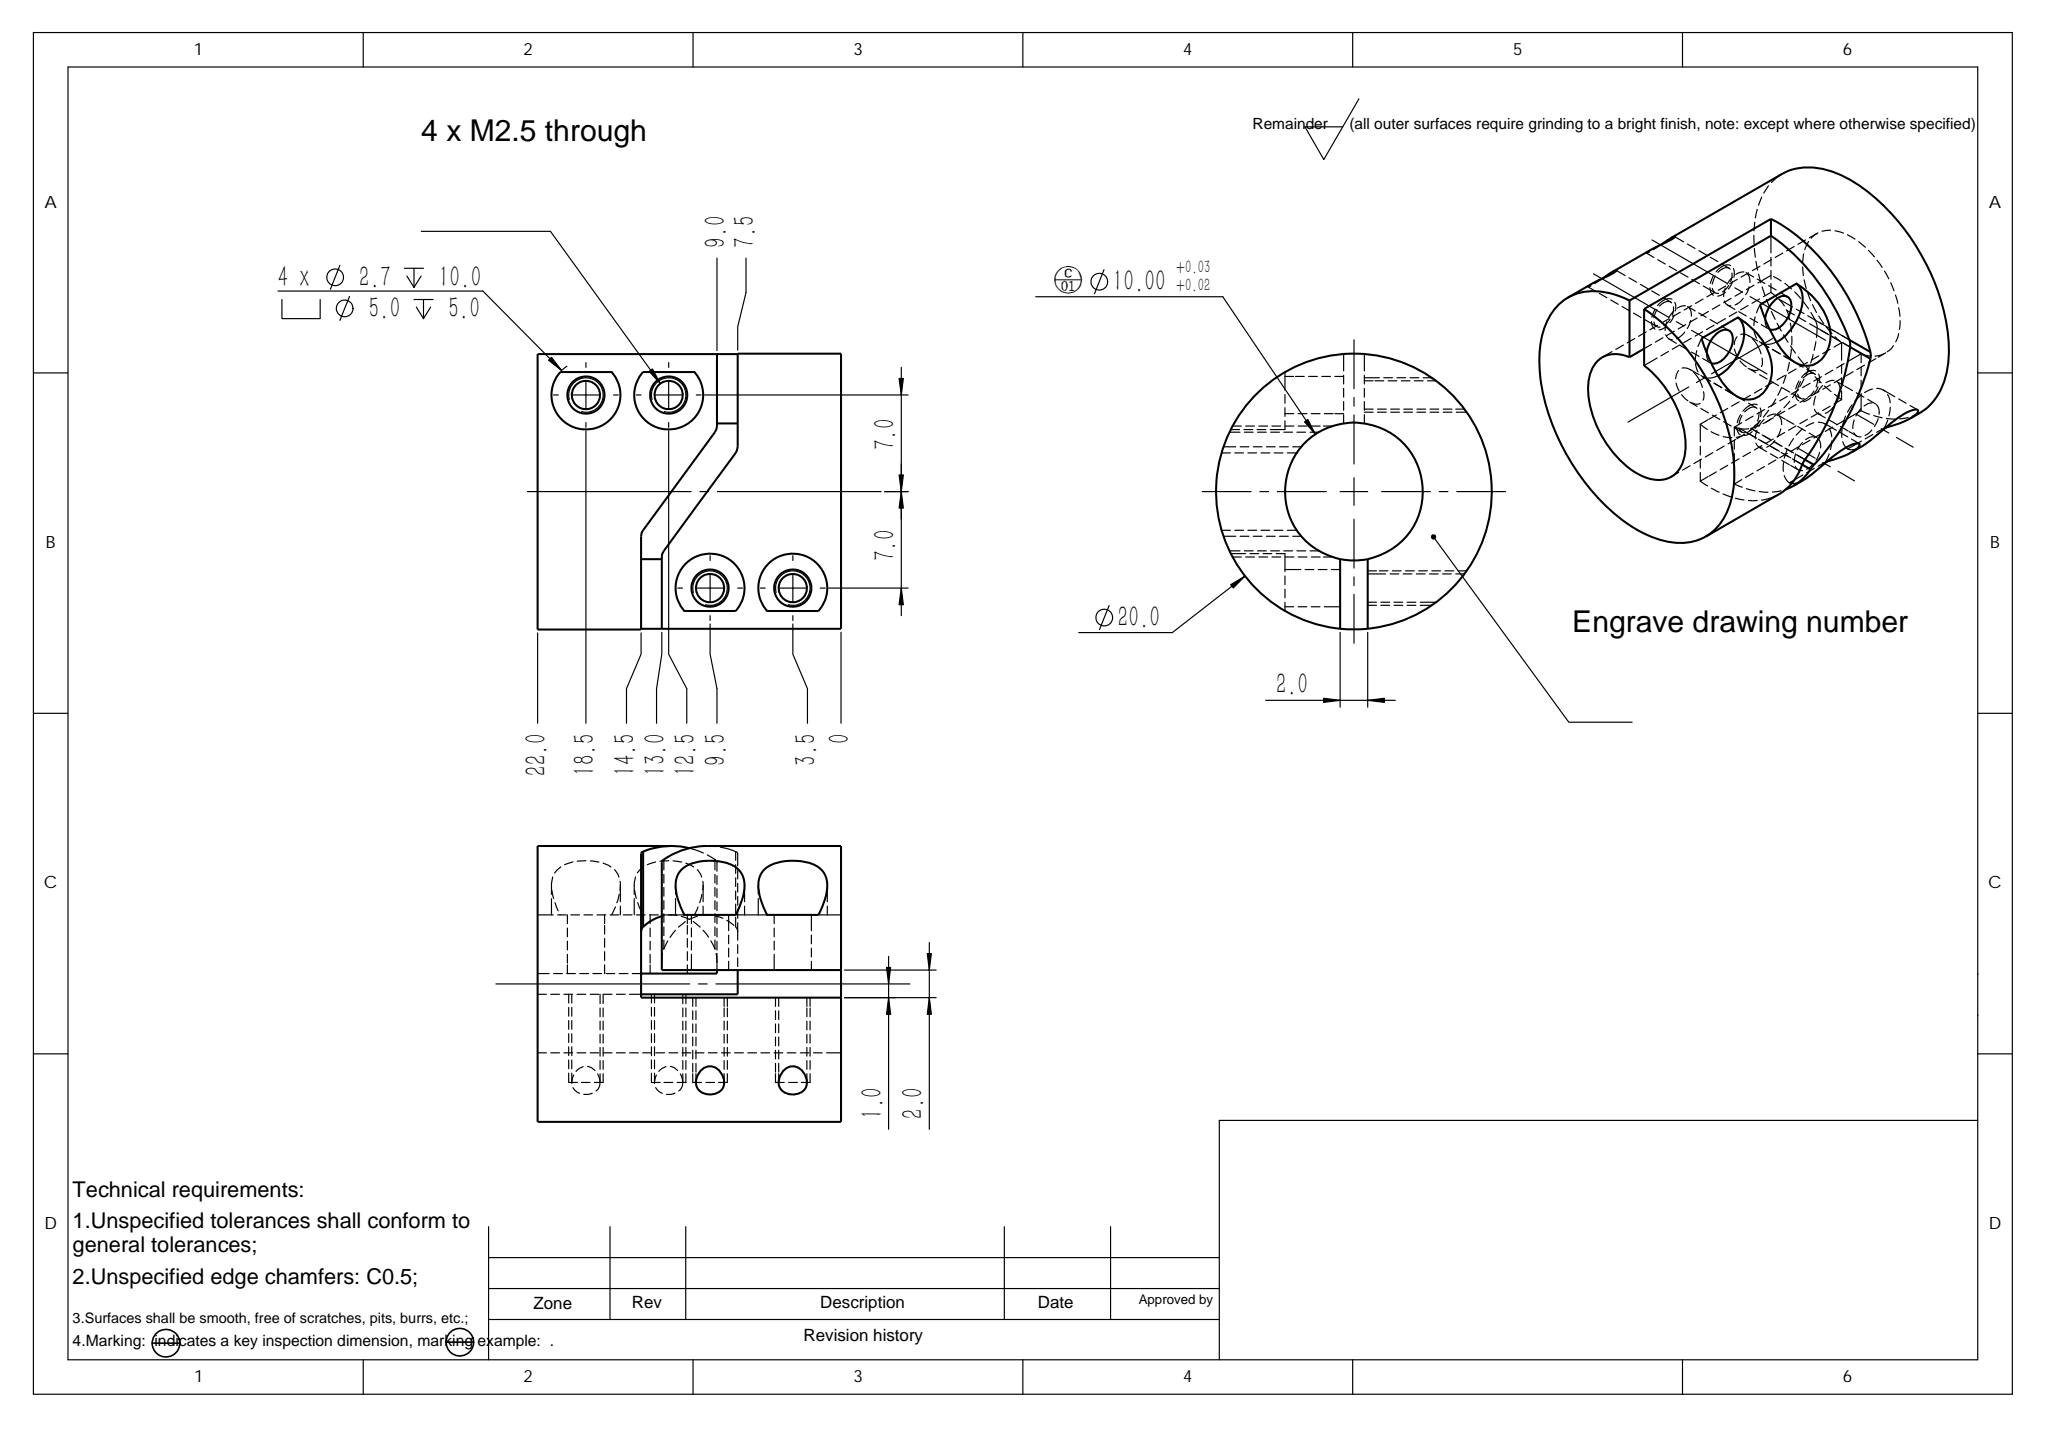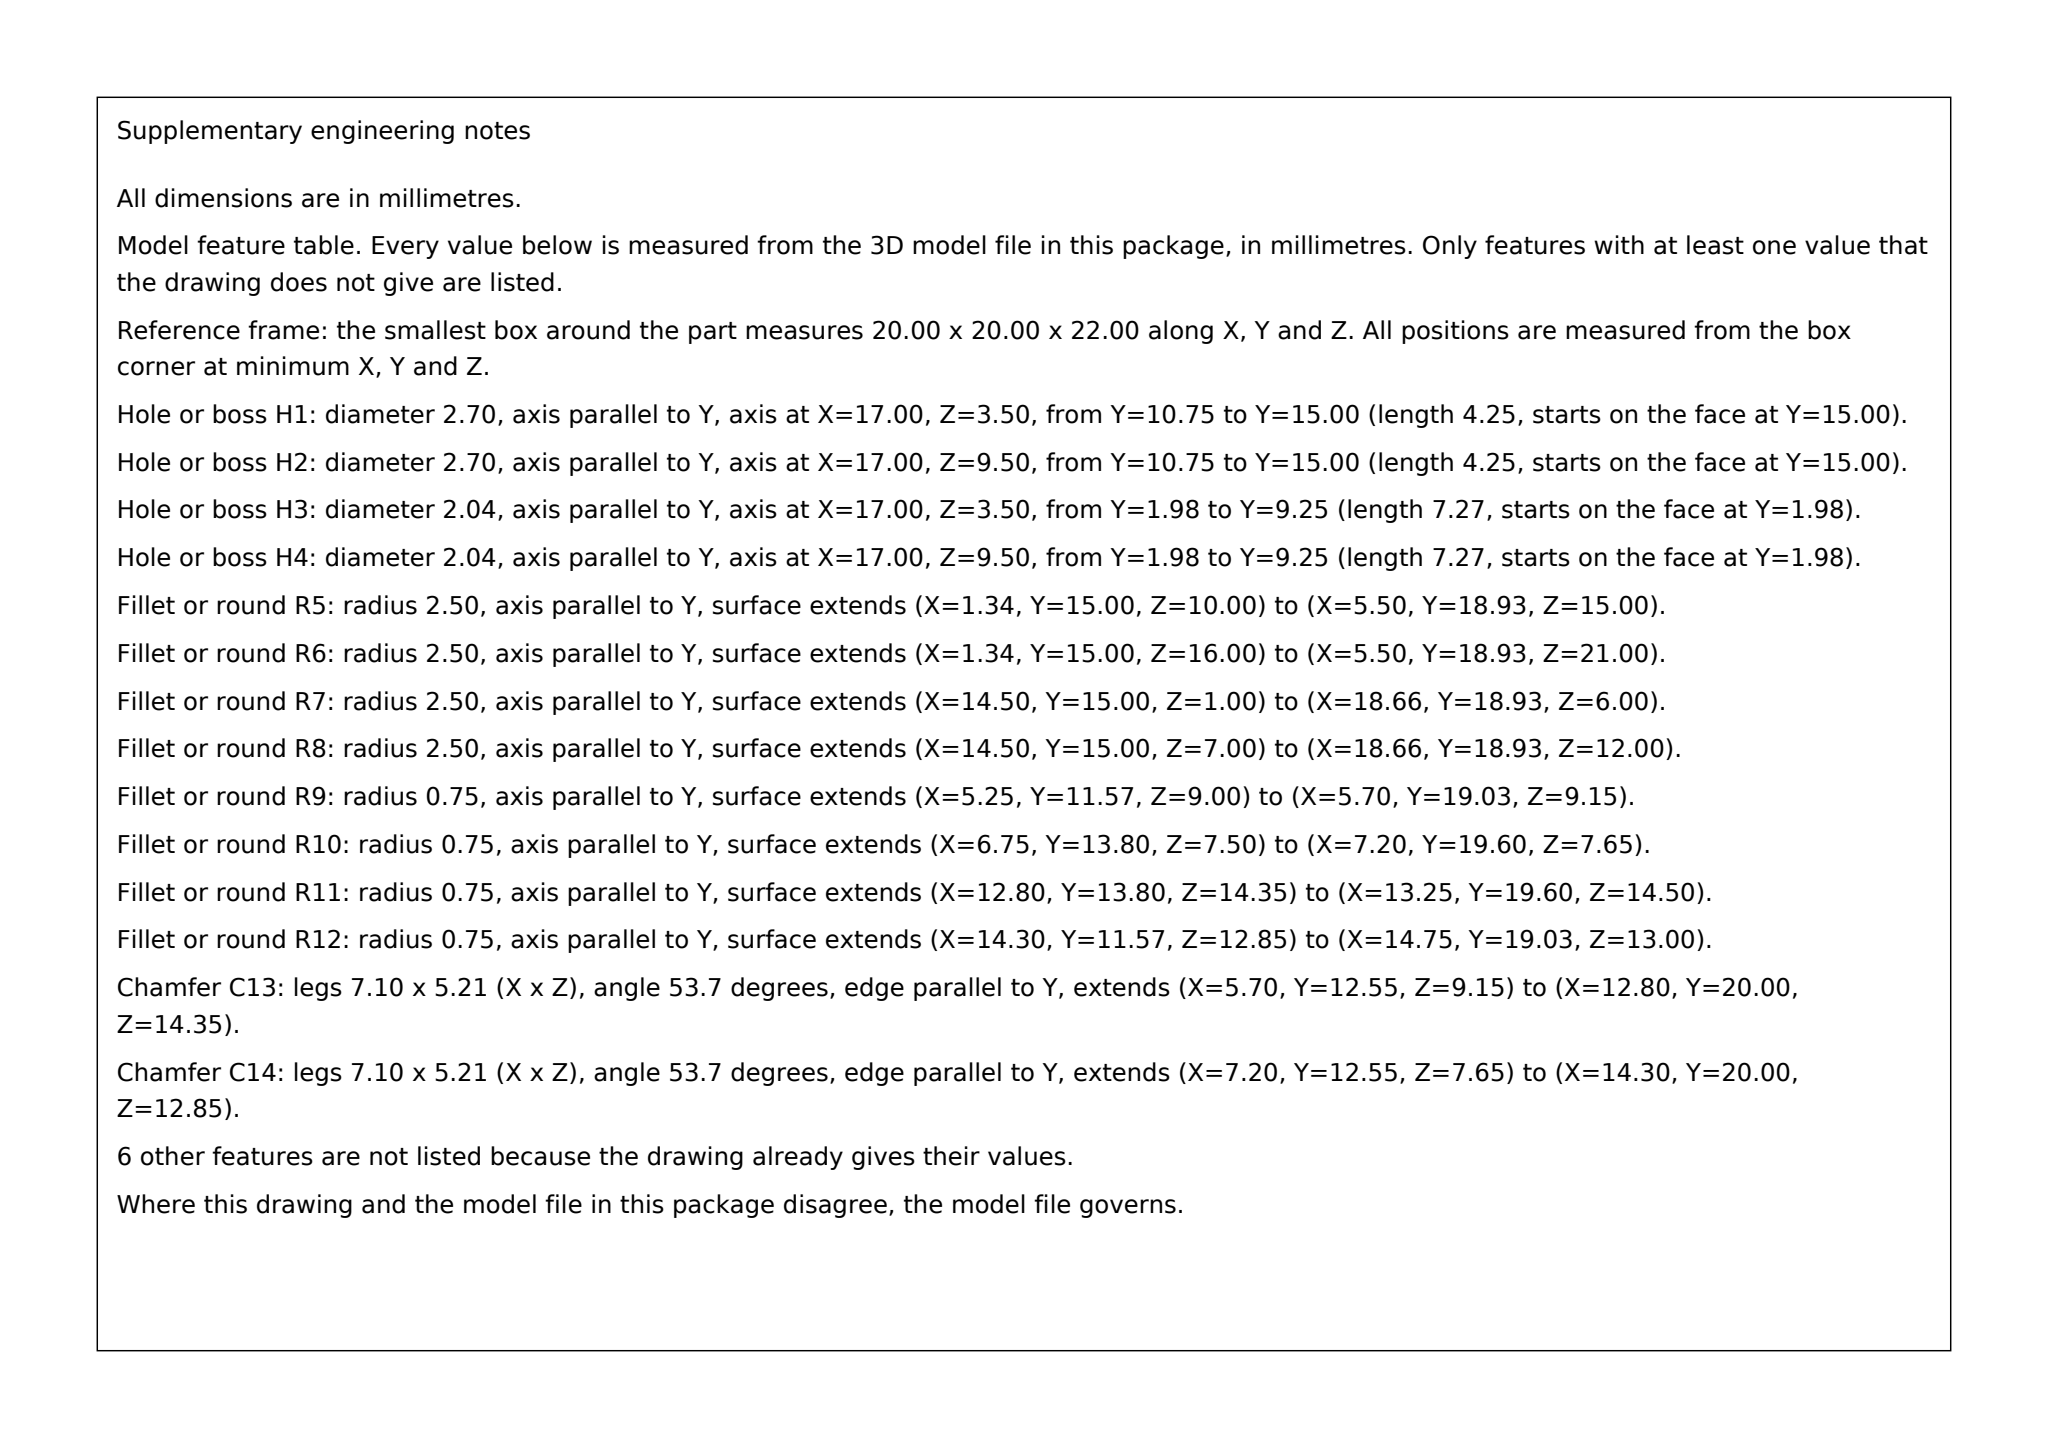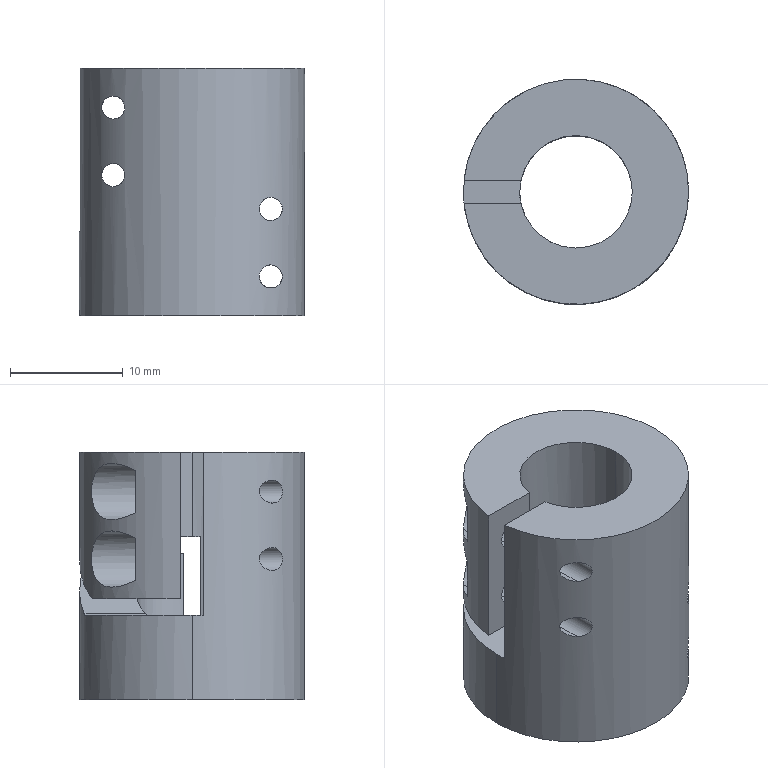Part | SolidWorks | mm | 1 solid | 54 faces | box 20 x 20 x 22 mm | volume 4390 mm3 | cylinder 38 | plane 16 | commonest cylinder face diameters 5 x12 2.05 x8 2.7 x8 1.5 x4 10 x3 20 x3
Drawing notes:
BODY Ø20.0 X 22.0 LG, Ø10.0 BORE THRU | from the solid: Ø20 and Ø10 z-axis cyls on axis x=10,y=10, length 22.0; bbox z=22.0
2X FLAT 5.0 DP FROM Ø20 OD = 5.0 OFF BORE AXIS, FULL 22.0 LG | from the solid: axis_planes y=15.0 (4 faces) vs bore axis y=10 -> R10-5=5.0 deep; z faces only 0 and 22.0
2X STEP SLOT 1.5 WIDE, R0.75 ENDS, 45 DEG TO BORE AXIS; PAD STEP 45 DEG | from the solid: Ø1.5 y-axis cyls at 4 step corners; 1.5 gap between z planes 7.5/9.0 and 13.0/14.5; corners on x+z=15 and x+z=27
STEP SLOT FACES 7.5 & 9.0 AND 13.0 & 14.5 FROM LH END FACE | from the solid: axis_planes z=7.5, 9.0, 13.0, 14.5 with ends at z=0 and 22.0
SLIT 2.0 WIDE SYMM ABOUT BORE AXIS CL, 1.0 EA SIDE | from the solid: axis_planes y=9.0 and y=11.0 about bore axis y=10.0
4X M2.5 THRU PERP TO SLIT PLANE, 7.0 EA SIDE OF BORE AXIS | from the solid: Ø2.05 tap drills, axis y, at x=3.0 and x=17.0 vs bore axis x=10.0; slit normal is y
CBORE Ø5.0 DP 5.0 & Ø2.7 DP 10.0 FROM FLAT FACE | from the solid: Ø5.0 and Ø2.7 y-axis cyls start at flat plane y=15.0; 15.0-5.0=10.0 = slit face
2X STEP SLOT END-HOLE CENTRES (R0.75 ENDS): OFFSET 3.25 AND 4.75 FROM BORE AXIS IN X; LH SLOT AT Z 8.25 & 9.75, RH SLOT AT Z 12.25 & 13.75 FROM LH END FACE | from the solid: Ø1.5 y-axis cylinders at (x5.25,z9.75),(x6.75,z8.25),(x13.25,z13.75),(x14.75,z12.25); bore axis at x=10.0
2X STEP SLOT DEPTH MEASURED PERP TO FLAT FACE (FLAT 5.0 OFF BORE AXIS): 7.45 DP AT OUTER END, 5.8 DP AT INNER END | from the solid: Ø1.5 y-axis cylinder lengths 7.45 and 5.8 starting at flat plane y=15.0
STEP SLOT R0.75 END CENTRES 2.12 APART (1.5 IN X BY 1.5 IN Z, 45 DEG); OVERALL SLOT LENGTH 3.62 | from the solid: Ø1.5 end-hole centre pairs (5.25,9.75)-(6.75,8.25) and (13.25,13.75)-(14.75,12.25), slot width Ø1.5
2.0 WIDE SLIT: FACES AT 1.0 EA SIDE OF BORE AXIS, FULL 22.0 LG FROM LH END FACE (Z0) TO RH END FACE (Z22), CUT RADIALLY 5.0 DEEP FROM Ø20.0 OD INTO Ø10.0 BORE | from the solid: y-normal planes at 9.0 and 11.0 (bore axis y=10.0); end faces z=0.0 and z=22.0; Ø20.0 and Ø10.0 z-cylinders length 22.0
2X STEP SLOT, 1.5 WIDE (R0.75 ENDS): END-RADIUS CENTRES 4.75 AND 3.25 FROM BORE AXIS (X), AT 9.75/8.25 AND 13.75/12.25 FROM LH END FACE (Z) | from the solid: cylinders dia 1.5 axis y at (x,z) = (5.25,9.75),(6.75,8.25),(13.25,13.75),(14.75,12.25); bore axis at x=10.0; LH end face z=0.0
2X STEP SLOT DEPTH, PERP TO SLIT PLANE, FROM FLAT FACE: 7.45 AT DEEP END, 5.80 AT SHALLOW (STEP) END | from the solid: cylinders dia 1.5 axis y lengths 7.45 and 5.80 starting at flat plane y=15.0
STEP SLOT END-RADIUS CENTRE-TO-CENTRE 2.12 (1.5 X BY 1.5 Z, 45 DEG); OVERALL SLOT LENGTH 3.62 | from the solid: dia 1.5 y-axis cylinder pairs offset 1.5 in x and 1.5 in z (5.25,9.75)-(6.75,8.25) and (13.25,13.75)-(14.75,12.25)
build123d program:
from build123d import *

# Parameters (mm, degrees)
SKETCH1_R                                         = 10
SKETCH1_R_2                                       = 5
BOSS_EXTRUDE1_DEPTH                               = 11
SKETCH3_W                                         = 12
SKETCH3_H                                         = 2
CUT_EXTRUDE1_DEPTH                                = 14.5
SKETCH4_W                                         = 12
SKETCH4_H                                         = 1.5
CUT_EXTRUDE2_DEPTH                                = 13
CUT_EXTRUDE3_DEPTH                                = 15
M2_5_HEX_SOCKET_HEAD_CAP_SCREW_CBORE1_D           = 2.7
M2_5_HEX_SOCKET_HEAD_CAP_SCREW_CBORE1_DEPTH       = 10
M2_5_HEX_SOCKET_HEAD_CAP_SCREW_CBORE1_CBORE_D     = 5
M2_5_HEX_SOCKET_HEAD_CAP_SCREW_CBORE1_CBORE_DEPTH = 5
M2_5_HEX_SOCKET_HEAD_CAP_SCREW_CBORE1_TIP         = 0.8112
M2_5_TAPPED_HOLE1_D                               = 2.05
FILLET1_R                                         = 0.75


with BuildPart() as part:
    # Sketch1 → Boss-Extrude1 (new, symmetric)
    with BuildSketch(Plane.XY):
        Circle(SKETCH1_R)
        Circle(SKETCH1_R_2, mode=Mode.SUBTRACT)
    extrude(amount=BOSS_EXTRUDE1_DEPTH, both=True)

    # Sketch3 → Cut-Extrude1 (cut)
    with BuildSketch(Plane.XY.offset(11)):
        with Locations((-6, 0)):
            Rectangle(SKETCH3_W, SKETCH3_H)
    extrude(amount=-CUT_EXTRUDE1_DEPTH, mode=Mode.SUBTRACT)

    # Sketch4 → Cut-Extrude2 (cut)
    with BuildSketch(Plane(origin=(0, 0, -11), x_dir=(-1, 0, 0), z_dir=(0, 0, -1))):
        with Locations((-6, 0)):
            Rectangle(SKETCH4_W, SKETCH4_H)
    extrude(amount=-CUT_EXTRUDE2_DEPTH, mode=Mode.SUBTRACT)

    # Sketch5 → Cut-Extrude3 (cut)
    with BuildSketch(Plane(origin=(0, -0.75, 0), x_dir=(1, 0, 0), z_dir=(0, 1, 0))):
        Polygon((-10, 3.5), (-3, 3.5), (4.5, -2), (10, -2), (10, -3.5), (3, -3.5), (-4.5, 2), (-10, 2), align=None)
    extrude(amount=CUT_EXTRUDE3_DEPTH, mode=Mode.SUBTRACT)

    # M2.5 Hex Socket Head Cap Screw CBORE1
    with Locations(Plane(origin=(0, 10, 0), x_dir=(1, 0, 0), z_dir=(0, 1, 0))):
        with Locations((7, 1.5), (7, 7.5), (-7, -1.5), (-7, -7.5)):
            CounterBoreHole(M2_5_HEX_SOCKET_HEAD_CAP_SCREW_CBORE1_D / 2, M2_5_HEX_SOCKET_HEAD_CAP_SCREW_CBORE1_CBORE_D / 2, M2_5_HEX_SOCKET_HEAD_CAP_SCREW_CBORE1_CBORE_DEPTH, depth=M2_5_HEX_SOCKET_HEAD_CAP_SCREW_CBORE1_DEPTH)
            with Locations((0, 0, -(M2_5_HEX_SOCKET_HEAD_CAP_SCREW_CBORE1_DEPTH + M2_5_HEX_SOCKET_HEAD_CAP_SCREW_CBORE1_TIP / 2))):  # 118° drill point
                Cone(0, M2_5_HEX_SOCKET_HEAD_CAP_SCREW_CBORE1_D / 2, M2_5_HEX_SOCKET_HEAD_CAP_SCREW_CBORE1_TIP, mode=Mode.SUBTRACT)

    # M2.5 Tapped Hole1 (through all)
    with Locations(Plane(origin=(0, 0, 0), x_dir=(1, 0, 0), z_dir=(0, 1, 0))):
        with Locations((-7, -7.5), (-7, -1.5), (7, 1.5), (7, 7.5)):
            Hole(M2_5_TAPPED_HOLE1_D / 2)

    # Fillet1
    fillet1_edges = [part.edges().sort_by_distance(p)[0] for p in [
        (4.5, 5.555, 2),
        (-4.5, 5.555, -2),
        (-3, 6.77, -3.5),
        (3, 6.77, 3.5),
    ]]
    fillet(fillet1_edges, radius=FILLET1_R)


solid = part.part